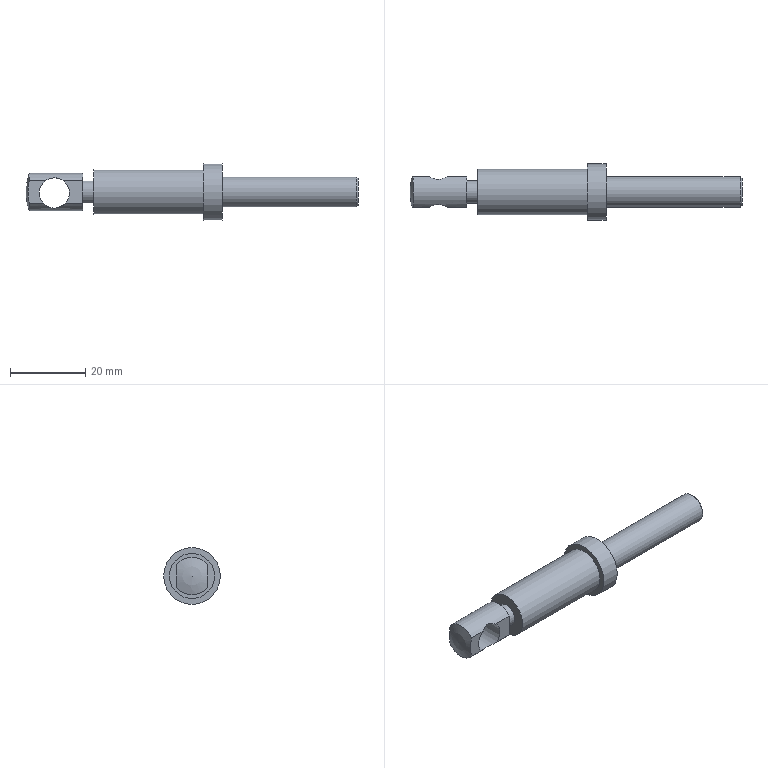Component | NX | CLHKJG_10_PISTON_ROD | 1 solid | 18 faces | volume 6687 mm3 | plane 9 | cylinder 7 | sphere 1 | cone 1 | commonest cylinder face diameters 10 x2 8 x2 12 x1 6 x1 15 x1